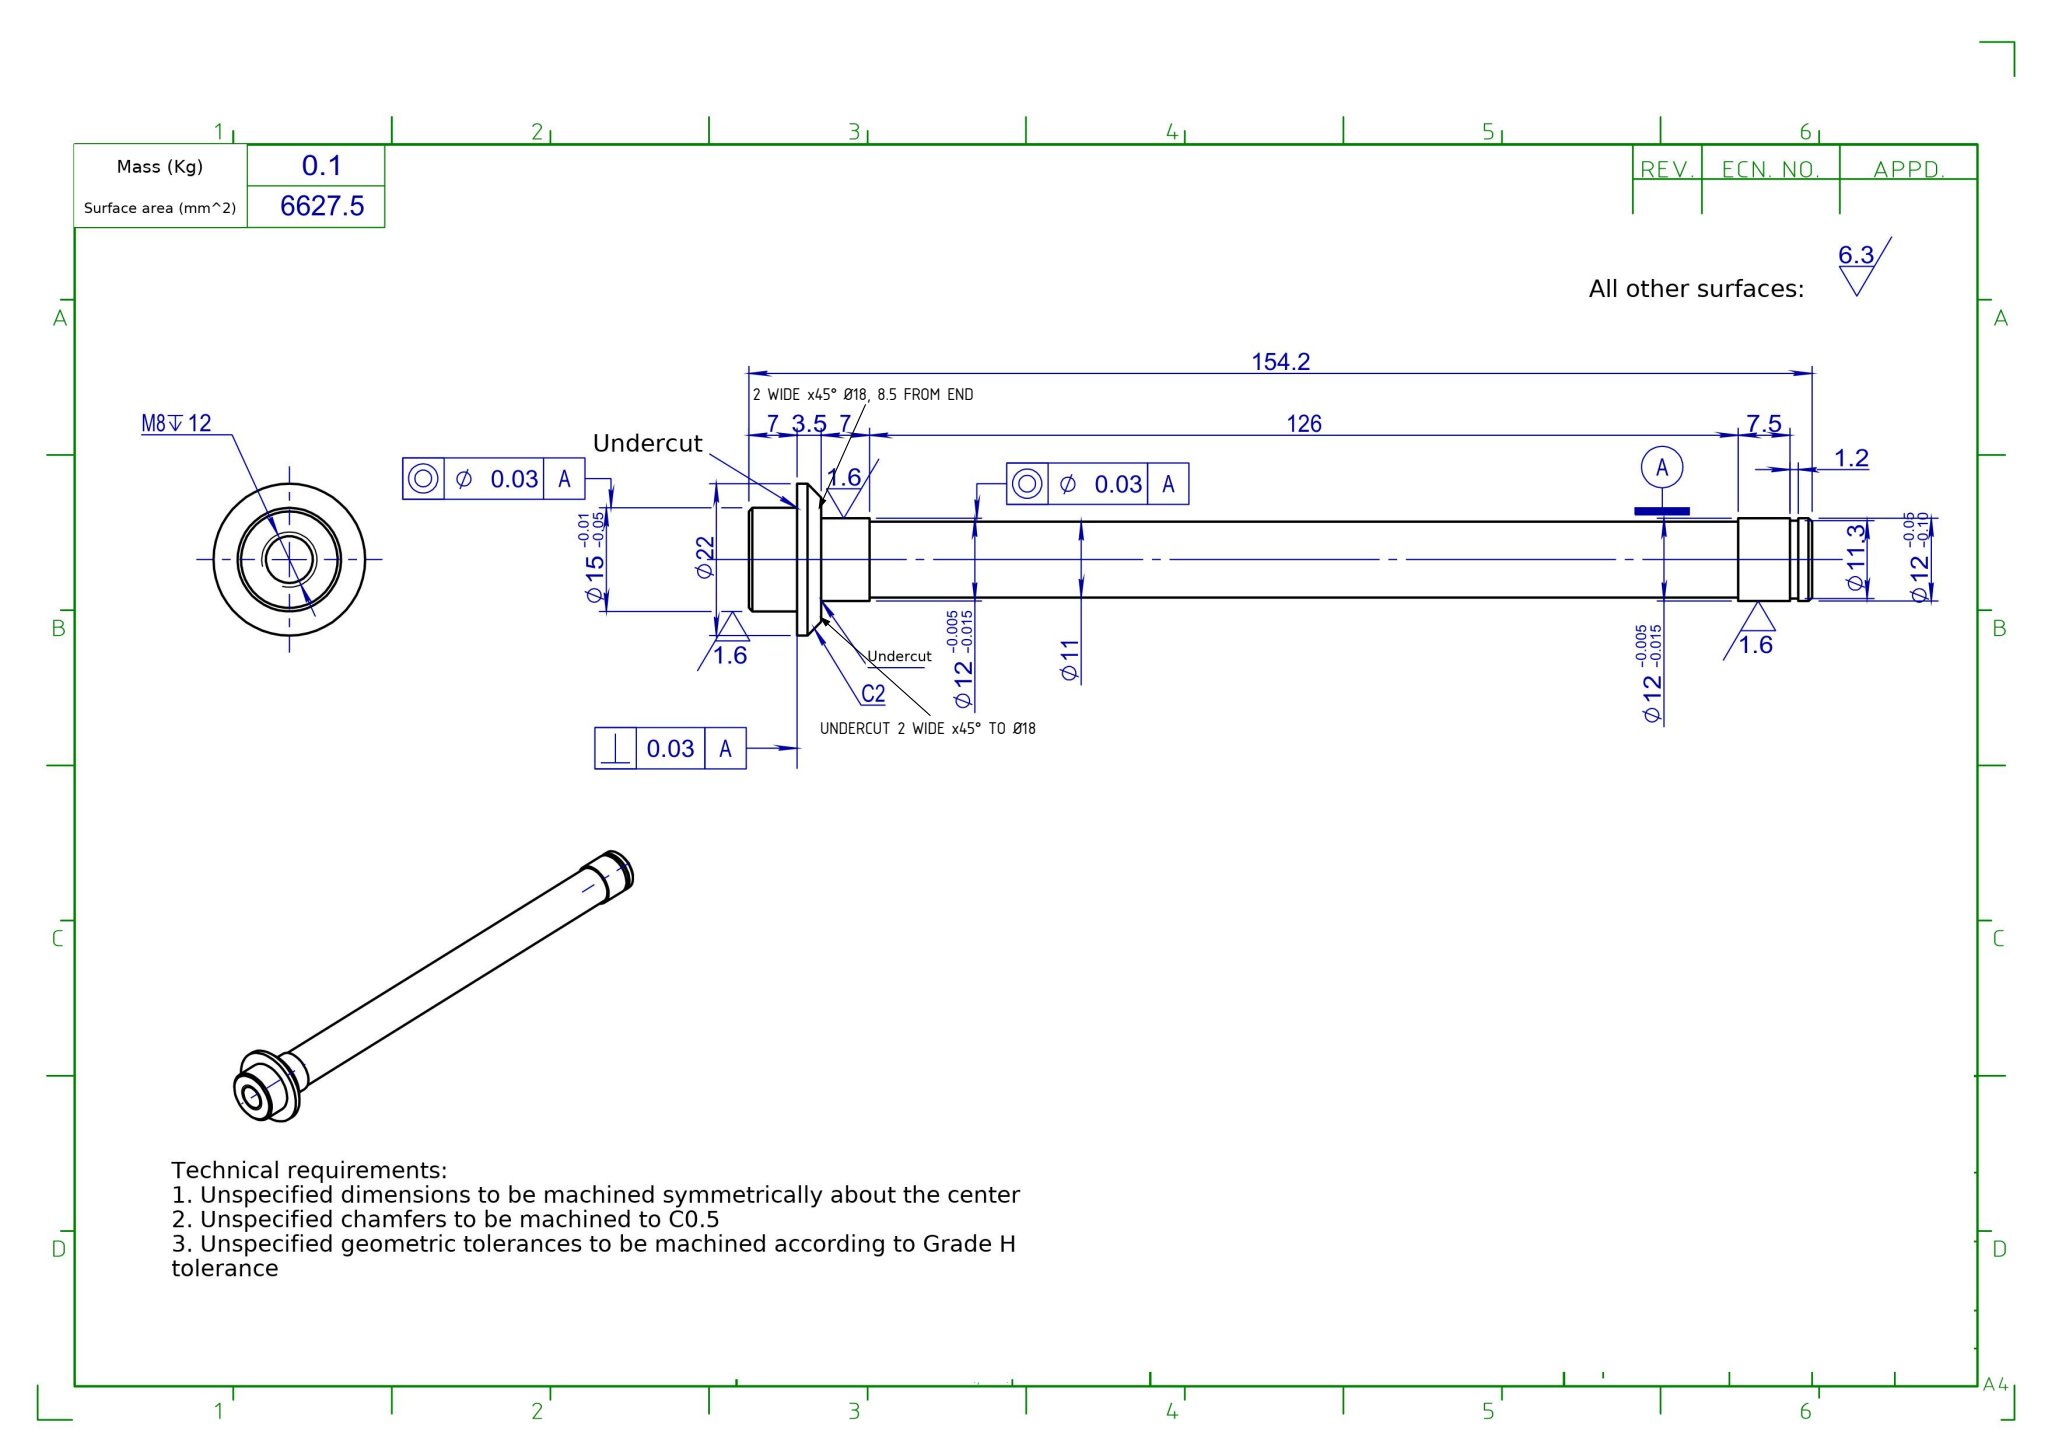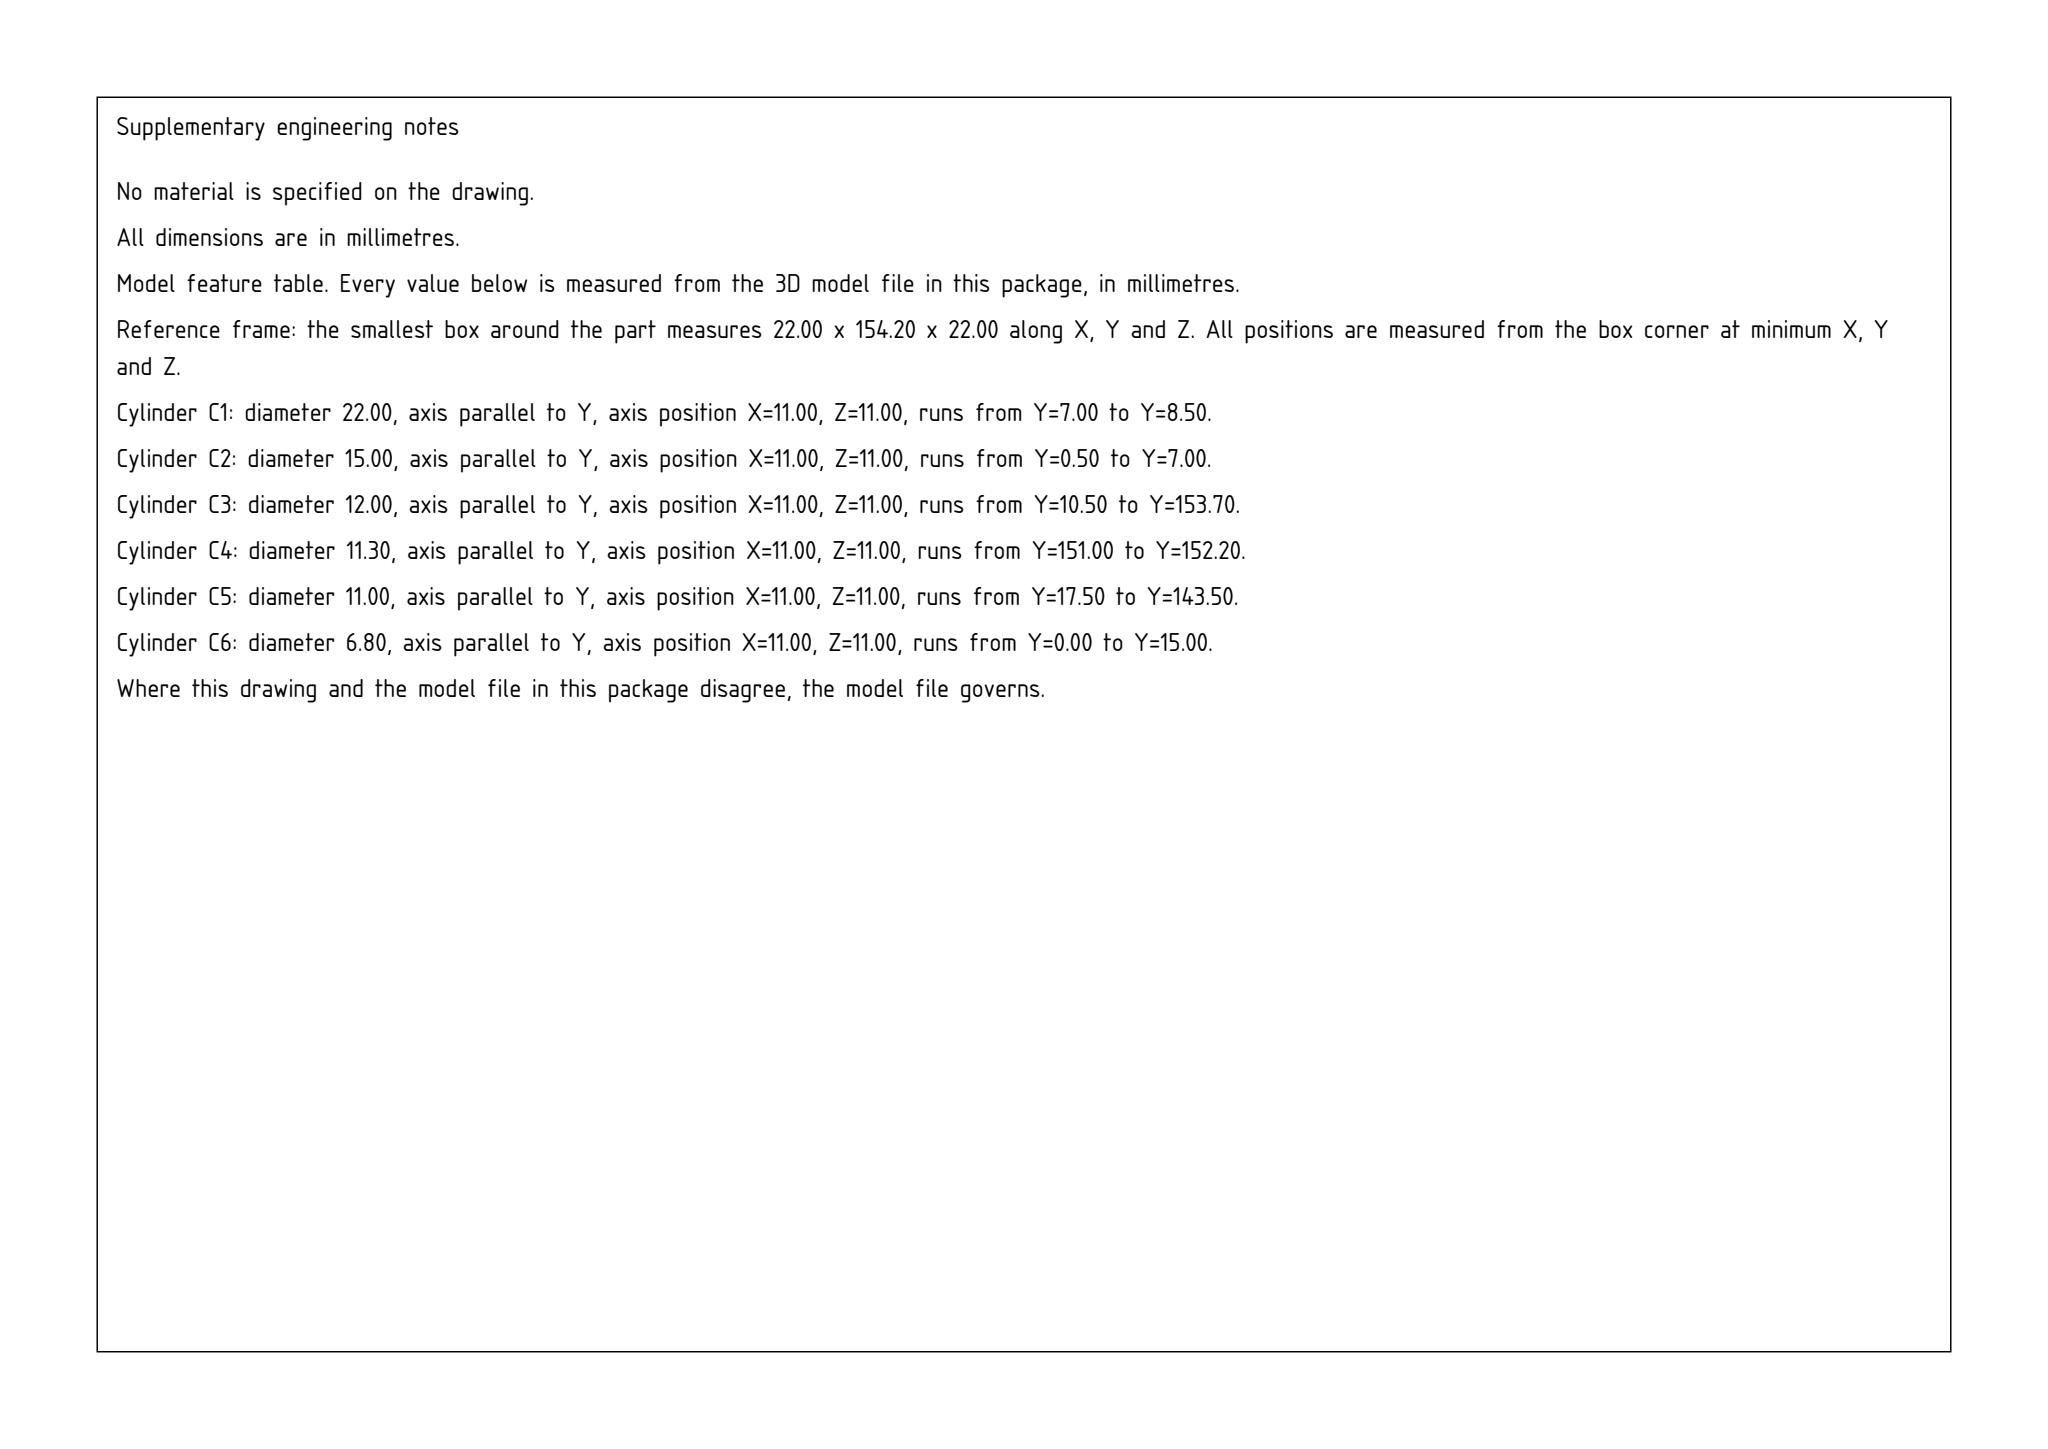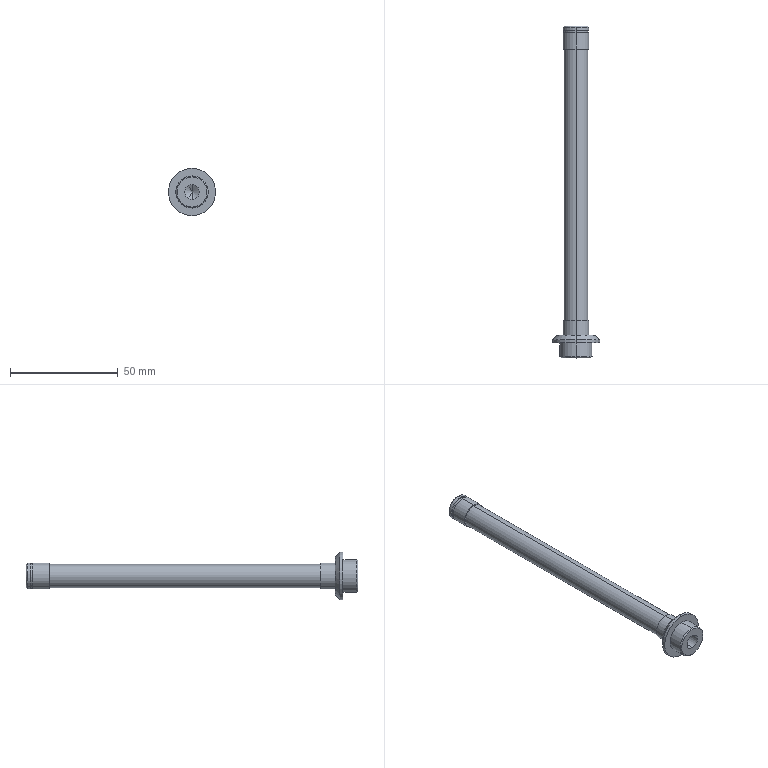Part | SolidWorks | mm | 1 solid | 32 faces | box 22 x 154.2 x 22 mm | volume 15818 mm3 | cylinder 16 | cone 8 | plane 8 | commonest cylinder face diameters 12 x6 6.8 x2 11.3 x2 11 x2 22 x2 15 x2
Drawing notes:
2ND UNDERCUT: 2 WIDE x 45° TO Ø18, STARTS 8.5 FROM LH END | from the solid: 90° cone (45° per side) ref dia 18, y 8.5->10.5, after Ø22 flange ending y=8.5; planar face y=10.5 spans Ø12 to Ø18
UNDERCUT AT Ø22 FLANGE: 2 WIDE x 45°, Ø18 ROOT, TO Ø12 SHLDR | from the solid: Ø22 flange y 7.0-8.5; cone 90° ref Ø18 y 8.5-10.5; Ø12 shaft starts y=10.5 (10.5 = 7 + 3.5 dim chain)
build123d program:
from build123d import *

# Parameters (mm, degrees)
SKETCH1_R             = 7.5
EXTRUDE1_DEPTH        = 7
SKETCH2_R             = 11
EXTRUDE2_DEPTH        = 3.5
SKETCH3_R             = 6
EXTRUDE3_DEPTH        = 7
SKETCH4_R             = 5.5
EXTRUDE4_DEPTH        = 126
SKETCH5_R             = 6
EXTRUDE5_DEPTH        = 7.5
SKETCH6_R             = 5.65
EXTRUDE6_DEPTH        = 1.2
SKETCH7_R             = 6
EXTRUDE7_DEPTH        = 2
M8_TAPPED_HOLE1_D     = 6.8
M8_TAPPED_HOLE1_DEPTH = 15
M8_TAPPED_HOLE1_TIP   = 2.043
CHAMFER1_SIZE         = 2
CHAMFER2_SIZE         = 0.5


with BuildPart() as part:
    # Sketch1 → Extrude1 (new body)
    with BuildSketch(Plane(origin=(0, 0, 0), x_dir=(1, 0, 0), z_dir=(0, 1, 0))):
        with Locations(Location((0, 0, 0), (0, 0, 270))):
            Circle(SKETCH1_R)
    extrude(amount=EXTRUDE1_DEPTH)

    # Sketch2 → Extrude2 (add)
    with BuildSketch(Plane(origin=(0, 7, 0), x_dir=(1, 0, 0), z_dir=(0, 1, 0))):
        with Locations(Location((0, 0, 0), (0, 0, 270))):
            Circle(SKETCH2_R)
    extrude(amount=EXTRUDE2_DEPTH)

    # Sketch3 → Extrude3 (add)
    with BuildSketch(Plane(origin=(0, 10.5, 0), x_dir=(1, 0, 0), z_dir=(0, 1, 0))):
        with Locations(Location((0, 0, 0), (0, 0, 270))):
            Circle(SKETCH3_R)
    extrude(amount=EXTRUDE3_DEPTH)

    # Sketch4 → Extrude4 (add)
    with BuildSketch(Plane(origin=(0, 17.5, 0), x_dir=(1, 0, 0), z_dir=(0, 1, 0))):
        with Locations(Location((0, 0, 0), (0, 0, 270))):
            Circle(SKETCH4_R)
    extrude(amount=EXTRUDE4_DEPTH)

    # Sketch5 → Extrude5 (add)
    with BuildSketch(Plane(origin=(0, 143.5, 0), x_dir=(1, 0, 0), z_dir=(0, 1, 0))):
        with Locations(Location((0, 0, 0), (0, 0, 270))):
            Circle(SKETCH5_R)
    extrude(amount=EXTRUDE5_DEPTH)

    # Sketch6 → Extrude6 (add)
    with BuildSketch(Plane(origin=(0, 151, 0), x_dir=(1, 0, 0), z_dir=(0, 1, 0))):
        with Locations(Location((0, 0, 0), (0, 0, 270))):
            Circle(SKETCH6_R)
    extrude(amount=EXTRUDE6_DEPTH)

    # Sketch7 → Extrude7 (add)
    with BuildSketch(Plane(origin=(0, 152.2, 0), x_dir=(1, 0, 0), z_dir=(0, 1, 0))):
        with Locations(Location((0, 0, 0), (0, 0, 270))):
            Circle(SKETCH7_R)
    extrude(amount=EXTRUDE7_DEPTH)

    # M8 Tapped Hole1
    with Locations(Plane.XZ):
        with Locations((0, 0)):
            Hole(M8_TAPPED_HOLE1_D / 2, depth=M8_TAPPED_HOLE1_DEPTH)
            with Locations((0, 0, -(M8_TAPPED_HOLE1_DEPTH + M8_TAPPED_HOLE1_TIP / 2))):  # 118° drill point
                Cone(0, M8_TAPPED_HOLE1_D / 2, M8_TAPPED_HOLE1_TIP, mode=Mode.SUBTRACT)

    # Chamfer1
    chamfer1_edges = [part.edges().sort_by_distance(p)[0] for p in [
        (0, 10.5, -11),
    ]]
    chamfer(chamfer1_edges, length=CHAMFER1_SIZE)

    # Chamfer2
    chamfer2_edges = [part.edges().sort_by_distance(p)[0] for p in [
        (0, 0, -7.5),
        (0, 154.2, -6),
    ]]
    chamfer(chamfer2_edges, length=CHAMFER2_SIZE)


solid = part.part
STEP:
#1=CARTESIAN_POINT('',(0.,0.,-7.));
#2=VERTEX_POINT('',#1);
#3=CARTESIAN_POINT('',(0.,0.,7.));
#4=VERTEX_POINT('',#3);
#5=CARTESIAN_POINT('',(0.,0.,0.));
#6=DIRECTION('',(0.,-1.,0.));
#7=DIRECTION('',(0.,0.,1.));
#8=AXIS2_PLACEMENT_3D('',#5,#6,#7);
#9=CIRCLE('',#8,7.);
#10=EDGE_CURVE('',#2,#4,#9,.T.);
#11=ORIENTED_EDGE('',*,*,#10,.F.);
#12=CARTESIAN_POINT('',(0.,0.5,-7.5));
#13=VERTEX_POINT('',#12);
#14=CARTESIAN_POINT('',(0.,0.5,-7.5));
#15=DIRECTION('',(0.,0.7071,-0.7071));
#16=VECTOR('',#15,1000.);
#17=LINE('',#14,#16);
#18=EDGE_CURVE('',#2,#13,#17,.T.);
#19=ORIENTED_EDGE('',*,*,#18,.T.);
#20=CARTESIAN_POINT('',(0.,0.5,7.5));
#21=VERTEX_POINT('',#20);
#22=CARTESIAN_POINT('',(0.,0.5,0.));
#23=DIRECTION('',(0.,1.,0.));
#24=DIRECTION('',(0.,0.,1.));
#25=AXIS2_PLACEMENT_3D('',#22,#23,#24);
#26=CIRCLE('',#25,7.5);
#27=EDGE_CURVE('',#21,#13,#26,.T.);
#28=ORIENTED_EDGE('',*,*,#27,.F.);
#29=CARTESIAN_POINT('',(0.,0.5,7.5));
#30=DIRECTION('',(0.,0.7071,0.7071));
#31=VECTOR('',#30,1000.);
#32=LINE('',#29,#31);
#33=EDGE_CURVE('',#4,#21,#32,.T.);
#34=ORIENTED_EDGE('',*,*,#33,.F.);
#35=EDGE_LOOP('',(#11,#19,#28,#34));
#36=FACE_OUTER_BOUND('',#35,.T.);
#37=CARTESIAN_POINT('',(0.,0.5,0.));
#38=DIRECTION('',(0.,1.,0.));
#39=DIRECTION('',(0.,0.,1.));
#40=AXIS2_PLACEMENT_3D('',#37,#38,#39);
#41=CONICAL_SURFACE('',#40,7.5,0.7854);
#42=ADVANCED_FACE('',(#36),#41,.T.);
#43=CARTESIAN_POINT('',(0.,154.2,5.5));
#44=VERTEX_POINT('',#43);
#45=CARTESIAN_POINT('',(0.,154.2,-5.5));
#46=VERTEX_POINT('',#45);
#47=CARTESIAN_POINT('',(0.,154.2,0.));
#48=DIRECTION('',(0.,1.,0.));
#49=DIRECTION('',(0.,0.,1.));
#50=AXIS2_PLACEMENT_3D('',#47,#48,#49);
#51=CIRCLE('',#50,5.5);
#52=EDGE_CURVE('',#44,#46,#51,.T.);
#53=ORIENTED_EDGE('',*,*,#52,.F.);
#54=CARTESIAN_POINT('',(0.,153.7,6.));
#55=VERTEX_POINT('',#54);
#56=CARTESIAN_POINT('',(0.,154.2,5.5));
#57=DIRECTION('',(0.,-0.7071,0.7071));
#58=VECTOR('',#57,1000.);
#59=LINE('',#56,#58);
#60=EDGE_CURVE('',#44,#55,#59,.T.);
#61=ORIENTED_EDGE('',*,*,#60,.T.);
#62=CARTESIAN_POINT('',(0.,153.7,-6.));
#63=VERTEX_POINT('',#62);
#64=CARTESIAN_POINT('',(0.,153.7,0.));
#65=DIRECTION('',(0.,-1.,0.));
#66=DIRECTION('',(0.,0.,1.));
#67=AXIS2_PLACEMENT_3D('',#64,#65,#66);
#68=CIRCLE('',#67,6.);
#69=EDGE_CURVE('',#63,#55,#68,.T.);
#70=ORIENTED_EDGE('',*,*,#69,.F.);
#71=CARTESIAN_POINT('',(0.,154.2,-5.5));
#72=DIRECTION('',(0.,-0.7071,-0.7071));
#73=VECTOR('',#72,1000.);
#74=LINE('',#71,#73);
#75=EDGE_CURVE('',#46,#63,#74,.T.);
#76=ORIENTED_EDGE('',*,*,#75,.F.);
#77=EDGE_LOOP('',(#53,#61,#70,#76));
#78=FACE_OUTER_BOUND('',#77,.T.);
#79=CARTESIAN_POINT('',(0.,154.2,0.));
#80=DIRECTION('',(0.,-1.,0.));
#81=DIRECTION('',(0.,0.,-1.));
#82=AXIS2_PLACEMENT_3D('',#79,#80,#81);
#83=CONICAL_SURFACE('',#82,5.5,0.7854);
#84=ADVANCED_FACE('',(#78),#83,.T.);
#85=CARTESIAN_POINT('',(0.,10.5,9.));
#86=VERTEX_POINT('',#85);
#87=CARTESIAN_POINT('',(0.,10.5,-9.));
#88=VERTEX_POINT('',#87);
#89=CARTESIAN_POINT('',(0.,10.5,0.));
#90=DIRECTION('',(0.,1.,0.));
#91=DIRECTION('',(0.,0.,1.));
#92=AXIS2_PLACEMENT_3D('',#89,#90,#91);
#93=CIRCLE('',#92,9.);
#94=EDGE_CURVE('',#86,#88,#93,.T.);
#95=ORIENTED_EDGE('',*,*,#94,.F.);
#96=CARTESIAN_POINT('',(0.,8.5,11.));
#97=VERTEX_POINT('',#96);
#98=CARTESIAN_POINT('',(0.,10.5,9.));
#99=DIRECTION('',(0.,-0.7071,0.7071));
#100=VECTOR('',#99,1000.);
#101=LINE('',#98,#100);
#102=EDGE_CURVE('',#86,#97,#101,.T.);
#103=ORIENTED_EDGE('',*,*,#102,.T.);
#104=CARTESIAN_POINT('',(0.,8.5,-11.));
#105=VERTEX_POINT('',#104);
#106=CARTESIAN_POINT('',(0.,8.5,0.));
#107=DIRECTION('',(0.,-1.,0.));
#108=DIRECTION('',(0.,0.,1.));
#109=AXIS2_PLACEMENT_3D('',#106,#107,#108);
#110=CIRCLE('',#109,11.);
#111=EDGE_CURVE('',#105,#97,#110,.T.);
#112=ORIENTED_EDGE('',*,*,#111,.F.);
#113=CARTESIAN_POINT('',(0.,10.5,-9.));
#114=DIRECTION('',(0.,-0.7071,-0.7071));
#115=VECTOR('',#114,1000.);
#116=LINE('',#113,#115);
#117=EDGE_CURVE('',#88,#105,#116,.T.);
#118=ORIENTED_EDGE('',*,*,#117,.F.);
#119=EDGE_LOOP('',(#95,#103,#112,#118));
#120=FACE_OUTER_BOUND('',#119,.T.);
#121=CARTESIAN_POINT('',(0.,10.5,0.));
#122=DIRECTION('',(0.,-1.,0.));
#123=DIRECTION('',(0.,0.,-1.));
#124=AXIS2_PLACEMENT_3D('',#121,#122,#123);
#125=CONICAL_SURFACE('',#124,9.,0.7854);
#126=ADVANCED_FACE('',(#120),#125,.T.);
#127=CARTESIAN_POINT('',(-0.,17.043,0.));
#128=VERTEX_POINT('',#127);
#129=CARTESIAN_POINT('',(0.,15.,-3.4));
#130=VERTEX_POINT('',#129);
#131=CARTESIAN_POINT('',(0.,15.,-3.4));
#132=DIRECTION('',(0.,-0.515,-0.8572));
#133=VECTOR('',#132,1000.);
#134=LINE('',#131,#133);
#135=EDGE_CURVE('',#128,#130,#134,.T.);
#136=ORIENTED_EDGE('',*,*,#135,.F.);
#137=CARTESIAN_POINT('',(0.,15.,3.4));
#138=VERTEX_POINT('',#137);
#139=CARTESIAN_POINT('',(0.,15.,3.4));
#140=DIRECTION('',(0.,-0.515,0.8572));
#141=VECTOR('',#140,1000.);
#142=LINE('',#139,#141);
#143=EDGE_CURVE('',#128,#138,#142,.T.);
#144=ORIENTED_EDGE('',*,*,#143,.T.);
#145=CARTESIAN_POINT('',(0.,15.,0.));
#146=DIRECTION('',(0.,-1.,0.));
#147=DIRECTION('',(0.,0.,-1.));
#148=AXIS2_PLACEMENT_3D('',#145,#146,#147);
#149=CIRCLE('',#148,3.4);
#150=EDGE_CURVE('',#138,#130,#149,.T.);
#151=ORIENTED_EDGE('',*,*,#150,.T.);
#152=EDGE_LOOP('',(#136,#144,#151));
#153=FACE_OUTER_BOUND('',#152,.T.);
#154=CARTESIAN_POINT('',(0.,15.,0.));
#155=DIRECTION('',(0.,-1.,0.));
#156=DIRECTION('',(0.,0.,-1.));
#157=AXIS2_PLACEMENT_3D('',#154,#155,#156);
#158=CONICAL_SURFACE('',#157,3.4,1.03);
#159=ADVANCED_FACE('',(#153),#158,.F.);
#160=ORIENTED_EDGE('',*,*,#150,.F.);
#161=CARTESIAN_POINT('',(0.,-0.,3.4));
#162=VERTEX_POINT('',#161);
#163=CARTESIAN_POINT('',(0.,0.,3.4));
#164=DIRECTION('',(0.,-1.,0.));
#165=VECTOR('',#164,1000.);
#166=LINE('',#163,#165);
#167=EDGE_CURVE('',#138,#162,#166,.T.);
#168=ORIENTED_EDGE('',*,*,#167,.T.);
#169=CARTESIAN_POINT('',(0.,-0.,-3.4));
#170=VERTEX_POINT('',#169);
#171=CARTESIAN_POINT('',(0.,-0.,0.));
#172=DIRECTION('',(0.,-1.,0.));
#173=DIRECTION('',(0.,0.,-1.));
#174=AXIS2_PLACEMENT_3D('',#171,#172,#173);
#175=CIRCLE('',#174,3.4);
#176=EDGE_CURVE('',#162,#170,#175,.T.);
#177=ORIENTED_EDGE('',*,*,#176,.T.);
#178=CARTESIAN_POINT('',(0.,0.,-3.4));
#179=DIRECTION('',(0.,-1.,0.));
#180=VECTOR('',#179,1000.);
#181=LINE('',#178,#180);
#182=EDGE_CURVE('',#130,#170,#181,.T.);
#183=ORIENTED_EDGE('',*,*,#182,.F.);
#184=EDGE_LOOP('',(#160,#168,#177,#183));
#185=FACE_OUTER_BOUND('',#184,.T.);
#186=CARTESIAN_POINT('',(0.,0.,0.));
#187=DIRECTION('',(0.,-1.,0.));
#188=DIRECTION('',(0.,0.,-1.));
#189=AXIS2_PLACEMENT_3D('',#186,#187,#188);
#190=CYLINDRICAL_SURFACE('',#189,3.4);
#191=ADVANCED_FACE('',(#185),#190,.F.);
#192=ORIENTED_EDGE('',*,*,#69,.T.);
#193=CARTESIAN_POINT('',(0.,152.2,6.));
#194=VERTEX_POINT('',#193);
#195=CARTESIAN_POINT('',(0.,154.2,6.));
#196=DIRECTION('',(0.,-1.,0.));
#197=VECTOR('',#196,1000.);
#198=LINE('',#195,#197);
#199=EDGE_CURVE('',#55,#194,#198,.T.);
#200=ORIENTED_EDGE('',*,*,#199,.T.);
#201=CARTESIAN_POINT('',(0.,152.2,-6.));
#202=VERTEX_POINT('',#201);
#203=CARTESIAN_POINT('',(0.,152.2,0.));
#204=DIRECTION('',(0.,1.,0.));
#205=DIRECTION('',(0.,0.,1.));
#206=AXIS2_PLACEMENT_3D('',#203,#204,#205);
#207=CIRCLE('',#206,6.);
#208=EDGE_CURVE('',#194,#202,#207,.T.);
#209=ORIENTED_EDGE('',*,*,#208,.T.);
#210=CARTESIAN_POINT('',(0.,154.2,-6.));
#211=DIRECTION('',(0.,-1.,0.));
#212=VECTOR('',#211,1000.);
#213=LINE('',#210,#212);
#214=EDGE_CURVE('',#63,#202,#213,.T.);
#215=ORIENTED_EDGE('',*,*,#214,.F.);
#216=EDGE_LOOP('',(#192,#200,#209,#215));
#217=FACE_OUTER_BOUND('',#216,.T.);
#218=CARTESIAN_POINT('',(0.,154.2,0.));
#219=DIRECTION('',(0.,-1.,0.));
#220=DIRECTION('',(0.,0.,-1.));
#221=AXIS2_PLACEMENT_3D('',#218,#219,#220);
#222=CYLINDRICAL_SURFACE('',#221,6.);
#223=ADVANCED_FACE('',(#217),#222,.T.);
#224=CARTESIAN_POINT('',(0.,152.2,5.65));
#225=VERTEX_POINT('',#224);
#226=CARTESIAN_POINT('',(0.,152.2,-5.65));
#227=VERTEX_POINT('',#226);
#228=CARTESIAN_POINT('',(0.,152.2,0.));
#229=DIRECTION('',(0.,1.,0.));
#230=DIRECTION('',(0.,0.,1.));
#231=AXIS2_PLACEMENT_3D('',#228,#229,#230);
#232=CIRCLE('',#231,5.65);
#233=EDGE_CURVE('',#225,#227,#232,.T.);
#234=ORIENTED_EDGE('',*,*,#233,.F.);
#235=CARTESIAN_POINT('',(0.,151.,5.65));
#236=VERTEX_POINT('',#235);
#237=CARTESIAN_POINT('',(0.,152.2,5.65));
#238=DIRECTION('',(0.,-1.,0.));
#239=VECTOR('',#238,1000.);
#240=LINE('',#237,#239);
#241=EDGE_CURVE('',#225,#236,#240,.T.);
#242=ORIENTED_EDGE('',*,*,#241,.T.);
#243=CARTESIAN_POINT('',(0.,151.,-5.65));
#244=VERTEX_POINT('',#243);
#245=CARTESIAN_POINT('',(0.,151.,0.));
#246=DIRECTION('',(0.,1.,0.));
#247=DIRECTION('',(0.,0.,1.));
#248=AXIS2_PLACEMENT_3D('',#245,#246,#247);
#249=CIRCLE('',#248,5.65);
#250=EDGE_CURVE('',#236,#244,#249,.T.);
#251=ORIENTED_EDGE('',*,*,#250,.T.);
#252=CARTESIAN_POINT('',(0.,152.2,-5.65));
#253=DIRECTION('',(0.,-1.,0.));
#254=VECTOR('',#253,1000.);
#255=LINE('',#252,#254);
#256=EDGE_CURVE('',#227,#244,#255,.T.);
#257=ORIENTED_EDGE('',*,*,#256,.F.);
#258=EDGE_LOOP('',(#234,#242,#251,#257));
#259=FACE_OUTER_BOUND('',#258,.T.);
#260=CARTESIAN_POINT('',(0.,152.2,0.));
#261=DIRECTION('',(0.,-1.,0.));
#262=DIRECTION('',(0.,0.,-1.));
#263=AXIS2_PLACEMENT_3D('',#260,#261,#262);
#264=CYLINDRICAL_SURFACE('',#263,5.65);
#265=ADVANCED_FACE('',(#259),#264,.T.);
#266=CARTESIAN_POINT('',(0.,151.,6.));
#267=VERTEX_POINT('',#266);
#268=CARTESIAN_POINT('',(0.,151.,-6.));
#269=VERTEX_POINT('',#268);
#270=CARTESIAN_POINT('',(0.,151.,0.));
#271=DIRECTION('',(0.,1.,0.));
#272=DIRECTION('',(0.,0.,1.));
#273=AXIS2_PLACEMENT_3D('',#270,#271,#272);
#274=CIRCLE('',#273,6.);
#275=EDGE_CURVE('',#267,#269,#274,.T.);
#276=ORIENTED_EDGE('',*,*,#275,.F.);
#277=CARTESIAN_POINT('',(0.,143.5,6.));
#278=VERTEX_POINT('',#277);
#279=CARTESIAN_POINT('',(0.,151.,6.));
#280=DIRECTION('',(0.,-1.,0.));
#281=VECTOR('',#280,1000.);
#282=LINE('',#279,#281);
#283=EDGE_CURVE('',#267,#278,#282,.T.);
#284=ORIENTED_EDGE('',*,*,#283,.T.);
#285=CARTESIAN_POINT('',(0.,143.5,-6.));
#286=VERTEX_POINT('',#285);
#287=CARTESIAN_POINT('',(0.,143.5,0.));
#288=DIRECTION('',(0.,1.,0.));
#289=DIRECTION('',(0.,0.,1.));
#290=AXIS2_PLACEMENT_3D('',#287,#288,#289);
#291=CIRCLE('',#290,6.);
#292=EDGE_CURVE('',#278,#286,#291,.T.);
#293=ORIENTED_EDGE('',*,*,#292,.T.);
#294=CARTESIAN_POINT('',(0.,151.,-6.));
#295=DIRECTION('',(0.,-1.,0.));
#296=VECTOR('',#295,1000.);
#297=LINE('',#294,#296);
#298=EDGE_CURVE('',#269,#286,#297,.T.);
#299=ORIENTED_EDGE('',*,*,#298,.F.);
#300=EDGE_LOOP('',(#276,#284,#293,#299));
#301=FACE_OUTER_BOUND('',#300,.T.);
#302=CARTESIAN_POINT('',(0.,151.,0.));
#303=DIRECTION('',(0.,-1.,0.));
#304=DIRECTION('',(0.,0.,-1.));
#305=AXIS2_PLACEMENT_3D('',#302,#303,#304);
#306=CYLINDRICAL_SURFACE('',#305,6.);
#307=ADVANCED_FACE('',(#301),#306,.T.);
#308=CARTESIAN_POINT('',(0.,143.5,5.5));
#309=VERTEX_POINT('',#308);
#310=CARTESIAN_POINT('',(0.,143.5,-5.5));
#311=VERTEX_POINT('',#310);
#312=CARTESIAN_POINT('',(0.,143.5,0.));
#313=DIRECTION('',(0.,1.,0.));
#314=DIRECTION('',(0.,0.,1.));
#315=AXIS2_PLACEMENT_3D('',#312,#313,#314);
#316=CIRCLE('',#315,5.5);
#317=EDGE_CURVE('',#309,#311,#316,.T.);
#318=ORIENTED_EDGE('',*,*,#317,.F.);
#319=CARTESIAN_POINT('',(0.,17.5,5.5));
#320=VERTEX_POINT('',#319);
#321=CARTESIAN_POINT('',(0.,143.5,5.5));
#322=DIRECTION('',(0.,-1.,0.));
#323=VECTOR('',#322,1000.);
#324=LINE('',#321,#323);
#325=EDGE_CURVE('',#309,#320,#324,.T.);
#326=ORIENTED_EDGE('',*,*,#325,.T.);
#327=CARTESIAN_POINT('',(0.,17.5,-5.5));
#328=VERTEX_POINT('',#327);
#329=CARTESIAN_POINT('',(0.,17.5,0.));
#330=DIRECTION('',(0.,1.,0.));
#331=DIRECTION('',(0.,0.,1.));
#332=AXIS2_PLACEMENT_3D('',#329,#330,#331);
#333=CIRCLE('',#332,5.5);
#334=EDGE_CURVE('',#320,#328,#333,.T.);
#335=ORIENTED_EDGE('',*,*,#334,.T.);
#336=CARTESIAN_POINT('',(0.,143.5,-5.5));
#337=DIRECTION('',(0.,-1.,0.));
#338=VECTOR('',#337,1000.);
#339=LINE('',#336,#338);
#340=EDGE_CURVE('',#311,#328,#339,.T.);
#341=ORIENTED_EDGE('',*,*,#340,.F.);
#342=EDGE_LOOP('',(#318,#326,#335,#341));
#343=FACE_OUTER_BOUND('',#342,.T.);
#344=CARTESIAN_POINT('',(0.,143.5,0.));
#345=DIRECTION('',(0.,-1.,0.));
#346=DIRECTION('',(0.,0.,-1.));
#347=AXIS2_PLACEMENT_3D('',#344,#345,#346);
#348=CYLINDRICAL_SURFACE('',#347,5.5);
#349=ADVANCED_FACE('',(#343),#348,.T.);
#350=CARTESIAN_POINT('',(0.,17.5,6.));
#351=VERTEX_POINT('',#350);
#352=CARTESIAN_POINT('',(0.,17.5,-6.));
#353=VERTEX_POINT('',#352);
#354=CARTESIAN_POINT('',(0.,17.5,0.));
#355=DIRECTION('',(0.,1.,0.));
#356=DIRECTION('',(0.,0.,1.));
#357=AXIS2_PLACEMENT_3D('',#354,#355,#356);
#358=CIRCLE('',#357,6.);
#359=EDGE_CURVE('',#351,#353,#358,.T.);
#360=ORIENTED_EDGE('',*,*,#359,.F.);
#361=CARTESIAN_POINT('',(0.,10.5,6.));
#362=VERTEX_POINT('',#361);
#363=CARTESIAN_POINT('',(0.,17.5,6.));
#364=DIRECTION('',(0.,-1.,0.));
#365=VECTOR('',#364,1000.);
#366=LINE('',#363,#365);
#367=EDGE_CURVE('',#351,#362,#366,.T.);
#368=ORIENTED_EDGE('',*,*,#367,.T.);
#369=CARTESIAN_POINT('',(0.,10.5,-6.));
#370=VERTEX_POINT('',#369);
#371=CARTESIAN_POINT('',(0.,10.5,0.));
#372=DIRECTION('',(0.,1.,0.));
#373=DIRECTION('',(0.,0.,1.));
#374=AXIS2_PLACEMENT_3D('',#371,#372,#373);
#375=CIRCLE('',#374,6.);
#376=EDGE_CURVE('',#362,#370,#375,.T.);
#377=ORIENTED_EDGE('',*,*,#376,.T.);
#378=CARTESIAN_POINT('',(0.,17.5,-6.));
#379=DIRECTION('',(0.,-1.,0.));
#380=VECTOR('',#379,1000.);
#381=LINE('',#378,#380);
#382=EDGE_CURVE('',#353,#370,#381,.T.);
#383=ORIENTED_EDGE('',*,*,#382,.F.);
#384=EDGE_LOOP('',(#360,#368,#377,#383));
#385=FACE_OUTER_BOUND('',#384,.T.);
#386=CARTESIAN_POINT('',(0.,17.5,0.));
#387=DIRECTION('',(0.,-1.,0.));
#388=DIRECTION('',(0.,0.,-1.));
#389=AXIS2_PLACEMENT_3D('',#386,#387,#388);
#390=CYLINDRICAL_SURFACE('',#389,6.);
#391=ADVANCED_FACE('',(#385),#390,.T.);
#392=ORIENTED_EDGE('',*,*,#111,.T.);
#393=CARTESIAN_POINT('',(0.,7.,11.));
#394=VERTEX_POINT('',#393);
#395=CARTESIAN_POINT('',(0.,10.5,11.));
#396=DIRECTION('',(0.,-1.,0.));
#397=VECTOR('',#396,1000.);
#398=LINE('',#395,#397);
#399=EDGE_CURVE('',#97,#394,#398,.T.);
#400=ORIENTED_EDGE('',*,*,#399,.T.);
#401=CARTESIAN_POINT('',(0.,7.,-11.));
#402=VERTEX_POINT('',#401);
#403=CARTESIAN_POINT('',(0.,7.,0.));
#404=DIRECTION('',(0.,1.,0.));
#405=DIRECTION('',(0.,0.,1.));
#406=AXIS2_PLACEMENT_3D('',#403,#404,#405);
#407=CIRCLE('',#406,11.);
#408=EDGE_CURVE('',#394,#402,#407,.T.);
#409=ORIENTED_EDGE('',*,*,#408,.T.);
#410=CARTESIAN_POINT('',(0.,10.5,-11.));
#411=DIRECTION('',(0.,-1.,0.));
#412=VECTOR('',#411,1000.);
#413=LINE('',#410,#412);
#414=EDGE_CURVE('',#105,#402,#413,.T.);
#415=ORIENTED_EDGE('',*,*,#414,.F.);
#416=EDGE_LOOP('',(#392,#400,#409,#415));
#417=FACE_OUTER_BOUND('',#416,.T.);
#418=CARTESIAN_POINT('',(0.,10.5,0.));
#419=DIRECTION('',(0.,-1.,0.));
#420=DIRECTION('',(0.,0.,-1.));
#421=AXIS2_PLACEMENT_3D('',#418,#419,#420);
#422=CYLINDRICAL_SURFACE('',#421,11.);
#423=ADVANCED_FACE('',(#417),#422,.T.);
#424=CARTESIAN_POINT('',(0.,7.,7.5));
#425=VERTEX_POINT('',#424);
#426=CARTESIAN_POINT('',(0.,7.,-7.5));
#427=VERTEX_POINT('',#426);
#428=CARTESIAN_POINT('',(0.,7.,0.));
#429=DIRECTION('',(0.,1.,0.));
#430=DIRECTION('',(0.,0.,1.));
#431=AXIS2_PLACEMENT_3D('',#428,#429,#430);
#432=CIRCLE('',#431,7.5);
#433=EDGE_CURVE('',#425,#427,#432,.T.);
#434=ORIENTED_EDGE('',*,*,#433,.F.);
#435=CARTESIAN_POINT('',(0.,7.,7.5));
#436=DIRECTION('',(0.,-1.,0.));
#437=VECTOR('',#436,1000.);
#438=LINE('',#435,#437);
#439=EDGE_CURVE('',#425,#21,#438,.T.);
#440=ORIENTED_EDGE('',*,*,#439,.T.);
#441=ORIENTED_EDGE('',*,*,#27,.T.);
#442=CARTESIAN_POINT('',(0.,7.,-7.5));
#443=DIRECTION('',(0.,-1.,0.));
#444=VECTOR('',#443,1000.);
#445=LINE('',#442,#444);
#446=EDGE_CURVE('',#427,#13,#445,.T.);
#447=ORIENTED_EDGE('',*,*,#446,.F.);
#448=EDGE_LOOP('',(#434,#440,#441,#447));
#449=FACE_OUTER_BOUND('',#448,.T.);
#450=CARTESIAN_POINT('',(0.,7.,0.));
#451=DIRECTION('',(0.,-1.,0.));
#452=DIRECTION('',(0.,0.,-1.));
#453=AXIS2_PLACEMENT_3D('',#450,#451,#452);
#454=CYLINDRICAL_SURFACE('',#453,7.5);
#455=ADVANCED_FACE('',(#449),#454,.T.);
#456=CARTESIAN_POINT('',(0.,151.,0.));
#457=DIRECTION('',(0.,1.,0.));
#458=DIRECTION('',(0.,0.,1.));
#459=AXIS2_PLACEMENT_3D('',#456,#457,#458);
#460=CIRCLE('',#459,6.);
#461=EDGE_CURVE('',#269,#267,#460,.T.);
#462=ORIENTED_EDGE('',*,*,#461,.T.);
#463=ORIENTED_EDGE('',*,*,#275,.T.);
#464=EDGE_LOOP('',(#462,#463));
#465=FACE_OUTER_BOUND('',#464,.T.);
#466=CARTESIAN_POINT('',(0.,151.,0.));
#467=DIRECTION('',(0.,1.,0.));
#468=DIRECTION('',(0.,0.,1.));
#469=AXIS2_PLACEMENT_3D('',#466,#467,#468);
#470=CIRCLE('',#469,5.65);
#471=EDGE_CURVE('',#244,#236,#470,.T.);
#472=ORIENTED_EDGE('',*,*,#471,.F.);
#473=ORIENTED_EDGE('',*,*,#250,.F.);
#474=EDGE_LOOP('',(#472,#473));
#475=FACE_BOUND('',#474,.T.);
#476=CARTESIAN_POINT('',(0.,151.,0.));
#477=DIRECTION('',(0.,1.,0.));
#478=DIRECTION('',(0.,0.,1.));
#479=AXIS2_PLACEMENT_3D('',#476,#477,#478);
#480=PLANE('',#479);
#481=ADVANCED_FACE('',(#465,#475),#480,.T.);
#482=CARTESIAN_POINT('',(0.,17.5,0.));
#483=DIRECTION('',(0.,1.,0.));
#484=DIRECTION('',(0.,0.,1.));
#485=AXIS2_PLACEMENT_3D('',#482,#483,#484);
#486=CIRCLE('',#485,6.);
#487=EDGE_CURVE('',#353,#351,#486,.T.);
#488=ORIENTED_EDGE('',*,*,#487,.T.);
#489=ORIENTED_EDGE('',*,*,#359,.T.);
#490=EDGE_LOOP('',(#488,#489));
#491=FACE_OUTER_BOUND('',#490,.T.);
#492=CARTESIAN_POINT('',(0.,17.5,0.));
#493=DIRECTION('',(0.,1.,0.));
#494=DIRECTION('',(0.,0.,1.));
#495=AXIS2_PLACEMENT_3D('',#492,#493,#494);
#496=CIRCLE('',#495,5.5);
#497=EDGE_CURVE('',#328,#320,#496,.T.);
#498=ORIENTED_EDGE('',*,*,#497,.F.);
#499=ORIENTED_EDGE('',*,*,#334,.F.);
#500=EDGE_LOOP('',(#498,#499));
#501=FACE_BOUND('',#500,.T.);
#502=CARTESIAN_POINT('',(0.,17.5,0.));
#503=DIRECTION('',(0.,1.,0.));
#504=DIRECTION('',(0.,0.,1.));
#505=AXIS2_PLACEMENT_3D('',#502,#503,#504);
#506=PLANE('',#505);
#507=ADVANCED_FACE('',(#491,#501),#506,.T.);
#508=CARTESIAN_POINT('',(0.,10.5,0.));
#509=DIRECTION('',(0.,1.,0.));
#510=DIRECTION('',(0.,0.,1.));
#511=AXIS2_PLACEMENT_3D('',#508,#509,#510);
#512=CIRCLE('',#511,9.);
#513=EDGE_CURVE('',#88,#86,#512,.T.);
#514=ORIENTED_EDGE('',*,*,#513,.T.);
#515=ORIENTED_EDGE('',*,*,#94,.T.);
#516=EDGE_LOOP('',(#514,#515));
#517=FACE_OUTER_BOUND('',#516,.T.);
#518=CARTESIAN_POINT('',(0.,10.5,0.));
#519=DIRECTION('',(0.,1.,0.));
#520=DIRECTION('',(0.,0.,1.));
#521=AXIS2_PLACEMENT_3D('',#518,#519,#520);
#522=CIRCLE('',#521,6.);
#523=EDGE_CURVE('',#370,#362,#522,.T.);
#524=ORIENTED_EDGE('',*,*,#523,.F.);
#525=ORIENTED_EDGE('',*,*,#376,.F.);
#526=EDGE_LOOP('',(#524,#525));
#527=FACE_BOUND('',#526,.T.);
#528=CARTESIAN_POINT('',(0.,10.5,0.));
#529=DIRECTION('',(0.,1.,0.));
#530=DIRECTION('',(0.,0.,1.));
#531=AXIS2_PLACEMENT_3D('',#528,#529,#530);
#532=PLANE('',#531);
#533=ADVANCED_FACE('',(#517,#527),#532,.T.);
#534=ORIENTED_EDGE('',*,*,#439,.F.);
#535=CARTESIAN_POINT('',(0.,7.,0.));
#536=DIRECTION('',(0.,1.,0.));
#537=DIRECTION('',(0.,0.,1.));
#538=AXIS2_PLACEMENT_3D('',#535,#536,#537);
#539=CIRCLE('',#538,7.5);
#540=EDGE_CURVE('',#427,#425,#539,.T.);
#541=ORIENTED_EDGE('',*,*,#540,.F.);
#542=ORIENTED_EDGE('',*,*,#446,.T.);
#543=CARTESIAN_POINT('',(0.,0.5,0.));
#544=DIRECTION('',(0.,1.,0.));
#545=DIRECTION('',(0.,0.,1.));
#546=AXIS2_PLACEMENT_3D('',#543,#544,#545);
#547=CIRCLE('',#546,7.5);
#548=EDGE_CURVE('',#13,#21,#547,.T.);
#549=ORIENTED_EDGE('',*,*,#548,.T.);
#550=EDGE_LOOP('',(#534,#541,#542,#549));
#551=FACE_OUTER_BOUND('',#550,.T.);
#552=CARTESIAN_POINT('',(0.,7.,0.));
#553=DIRECTION('',(0.,-1.,0.));
#554=DIRECTION('',(0.,0.,-1.));
#555=AXIS2_PLACEMENT_3D('',#552,#553,#554);
#556=CYLINDRICAL_SURFACE('',#555,7.5);
#557=ADVANCED_FACE('',(#551),#556,.T.);
#558=CARTESIAN_POINT('',(0.,0.,0.));
#559=DIRECTION('',(0.,-1.,0.));
#560=DIRECTION('',(0.,0.,1.));
#561=AXIS2_PLACEMENT_3D('',#558,#559,#560);
#562=CIRCLE('',#561,7.);
#563=EDGE_CURVE('',#4,#2,#562,.T.);
#564=ORIENTED_EDGE('',*,*,#563,.T.);
#565=ORIENTED_EDGE('',*,*,#10,.T.);
#566=EDGE_LOOP('',(#564,#565));
#567=FACE_OUTER_BOUND('',#566,.T.);
#568=CARTESIAN_POINT('',(0.,-0.,0.));
#569=DIRECTION('',(0.,-1.,0.));
#570=DIRECTION('',(0.,0.,-1.));
#571=AXIS2_PLACEMENT_3D('',#568,#569,#570);
#572=CIRCLE('',#571,3.4);
#573=EDGE_CURVE('',#170,#162,#572,.T.);
#574=ORIENTED_EDGE('',*,*,#573,.F.);
#575=ORIENTED_EDGE('',*,*,#176,.F.);
#576=EDGE_LOOP('',(#574,#575));
#577=FACE_BOUND('',#576,.T.);
#578=CARTESIAN_POINT('',(0.,0.,0.));
#579=DIRECTION('',(0.,1.,0.));
#580=DIRECTION('',(0.,0.,1.));
#581=AXIS2_PLACEMENT_3D('',#578,#579,#580);
#582=PLANE('',#581);
#583=ADVANCED_FACE('',(#567,#577),#582,.F.);
#584=CARTESIAN_POINT('',(0.,7.,0.));
#585=DIRECTION('',(0.,1.,0.));
#586=DIRECTION('',(0.,0.,1.));
#587=AXIS2_PLACEMENT_3D('',#584,#585,#586);
#588=CIRCLE('',#587,11.);
#589=EDGE_CURVE('',#402,#394,#588,.T.);
#590=ORIENTED_EDGE('',*,*,#589,.F.);
#591=ORIENTED_EDGE('',*,*,#408,.F.);
#592=EDGE_LOOP('',(#590,#591));
#593=FACE_OUTER_BOUND('',#592,.T.);
#594=ORIENTED_EDGE('',*,*,#540,.T.);
#595=ORIENTED_EDGE('',*,*,#433,.T.);
#596=EDGE_LOOP('',(#594,#595));
#597=FACE_BOUND('',#596,.T.);
#598=CARTESIAN_POINT('',(0.,7.,0.));
#599=DIRECTION('',(0.,1.,0.));
#600=DIRECTION('',(0.,0.,1.));
#601=AXIS2_PLACEMENT_3D('',#598,#599,#600);
#602=PLANE('',#601);
#603=ADVANCED_FACE('',(#593,#597),#602,.F.);
#604=ORIENTED_EDGE('',*,*,#399,.F.);
#605=CARTESIAN_POINT('',(0.,8.5,0.));
#606=DIRECTION('',(0.,-1.,0.));
#607=DIRECTION('',(0.,0.,1.));
#608=AXIS2_PLACEMENT_3D('',#605,#606,#607);
#609=CIRCLE('',#608,11.);
#610=EDGE_CURVE('',#97,#105,#609,.T.);
#611=ORIENTED_EDGE('',*,*,#610,.T.);
#612=ORIENTED_EDGE('',*,*,#414,.T.);
#613=ORIENTED_EDGE('',*,*,#589,.T.);
#614=EDGE_LOOP('',(#604,#611,#612,#613));
#615=FACE_OUTER_BOUND('',#614,.T.);
#616=CARTESIAN_POINT('',(0.,10.5,0.));
#617=DIRECTION('',(0.,-1.,0.));
#618=DIRECTION('',(0.,0.,-1.));
#619=AXIS2_PLACEMENT_3D('',#616,#617,#618);
#620=CYLINDRICAL_SURFACE('',#619,11.);
#621=ADVANCED_FACE('',(#615),#620,.T.);
#622=ORIENTED_EDGE('',*,*,#367,.F.);
#623=ORIENTED_EDGE('',*,*,#487,.F.);
#624=ORIENTED_EDGE('',*,*,#382,.T.);
#625=ORIENTED_EDGE('',*,*,#523,.T.);
#626=EDGE_LOOP('',(#622,#623,#624,#625));
#627=FACE_OUTER_BOUND('',#626,.T.);
#628=CARTESIAN_POINT('',(0.,17.5,0.));
#629=DIRECTION('',(0.,-1.,0.));
#630=DIRECTION('',(0.,0.,-1.));
#631=AXIS2_PLACEMENT_3D('',#628,#629,#630);
#632=CYLINDRICAL_SURFACE('',#631,6.);
#633=ADVANCED_FACE('',(#627),#632,.T.);
#634=ORIENTED_EDGE('',*,*,#325,.F.);
#635=CARTESIAN_POINT('',(0.,143.5,0.));
#636=DIRECTION('',(0.,1.,0.));
#637=DIRECTION('',(0.,0.,1.));
#638=AXIS2_PLACEMENT_3D('',#635,#636,#637);
#639=CIRCLE('',#638,5.5);
#640=EDGE_CURVE('',#311,#309,#639,.T.);
#641=ORIENTED_EDGE('',*,*,#640,.F.);
#642=ORIENTED_EDGE('',*,*,#340,.T.);
#643=ORIENTED_EDGE('',*,*,#497,.T.);
#644=EDGE_LOOP('',(#634,#641,#642,#643));
#645=FACE_OUTER_BOUND('',#644,.T.);
#646=CARTESIAN_POINT('',(0.,143.5,0.));
#647=DIRECTION('',(0.,-1.,0.));
#648=DIRECTION('',(0.,0.,-1.));
#649=AXIS2_PLACEMENT_3D('',#646,#647,#648);
#650=CYLINDRICAL_SURFACE('',#649,5.5);
#651=ADVANCED_FACE('',(#645),#650,.T.);
#652=CARTESIAN_POINT('',(0.,143.5,0.));
#653=DIRECTION('',(0.,1.,0.));
#654=DIRECTION('',(0.,0.,1.));
#655=AXIS2_PLACEMENT_3D('',#652,#653,#654);
#656=CIRCLE('',#655,6.);
#657=EDGE_CURVE('',#286,#278,#656,.T.);
#658=ORIENTED_EDGE('',*,*,#657,.F.);
#659=ORIENTED_EDGE('',*,*,#292,.F.);
#660=EDGE_LOOP('',(#658,#659));
#661=FACE_OUTER_BOUND('',#660,.T.);
#662=ORIENTED_EDGE('',*,*,#640,.T.);
#663=ORIENTED_EDGE('',*,*,#317,.T.);
#664=EDGE_LOOP('',(#662,#663));
#665=FACE_BOUND('',#664,.T.);
#666=CARTESIAN_POINT('',(0.,143.5,0.));
#667=DIRECTION('',(0.,1.,0.));
#668=DIRECTION('',(0.,0.,1.));
#669=AXIS2_PLACEMENT_3D('',#666,#667,#668);
#670=PLANE('',#669);
#671=ADVANCED_FACE('',(#661,#665),#670,.F.);
#672=ORIENTED_EDGE('',*,*,#283,.F.);
#673=ORIENTED_EDGE('',*,*,#461,.F.);
#674=ORIENTED_EDGE('',*,*,#298,.T.);
#675=ORIENTED_EDGE('',*,*,#657,.T.);
#676=EDGE_LOOP('',(#672,#673,#674,#675));
#677=FACE_OUTER_BOUND('',#676,.T.);
#678=CARTESIAN_POINT('',(0.,151.,0.));
#679=DIRECTION('',(0.,-1.,0.));
#680=DIRECTION('',(0.,0.,-1.));
#681=AXIS2_PLACEMENT_3D('',#678,#679,#680);
#682=CYLINDRICAL_SURFACE('',#681,6.);
#683=ADVANCED_FACE('',(#677),#682,.T.);
#684=ORIENTED_EDGE('',*,*,#241,.F.);
#685=CARTESIAN_POINT('',(0.,152.2,0.));
#686=DIRECTION('',(0.,1.,0.));
#687=DIRECTION('',(0.,0.,1.));
#688=AXIS2_PLACEMENT_3D('',#685,#686,#687);
#689=CIRCLE('',#688,5.65);
#690=EDGE_CURVE('',#227,#225,#689,.T.);
#691=ORIENTED_EDGE('',*,*,#690,.F.);
#692=ORIENTED_EDGE('',*,*,#256,.T.);
#693=ORIENTED_EDGE('',*,*,#471,.T.);
#694=EDGE_LOOP('',(#684,#691,#692,#693));
#695=FACE_OUTER_BOUND('',#694,.T.);
#696=CARTESIAN_POINT('',(0.,152.2,0.));
#697=DIRECTION('',(0.,-1.,0.));
#698=DIRECTION('',(0.,0.,-1.));
#699=AXIS2_PLACEMENT_3D('',#696,#697,#698);
#700=CYLINDRICAL_SURFACE('',#699,5.65);
#701=ADVANCED_FACE('',(#695),#700,.T.);
#702=CARTESIAN_POINT('',(0.,152.2,0.));
#703=DIRECTION('',(0.,1.,0.));
#704=DIRECTION('',(0.,0.,1.));
#705=AXIS2_PLACEMENT_3D('',#702,#703,#704);
#706=CIRCLE('',#705,6.);
#707=EDGE_CURVE('',#202,#194,#706,.T.);
#708=ORIENTED_EDGE('',*,*,#707,.F.);
#709=ORIENTED_EDGE('',*,*,#208,.F.);
#710=EDGE_LOOP('',(#708,#709));
#711=FACE_OUTER_BOUND('',#710,.T.);
#712=ORIENTED_EDGE('',*,*,#690,.T.);
#713=ORIENTED_EDGE('',*,*,#233,.T.);
#714=EDGE_LOOP('',(#712,#713));
#715=FACE_BOUND('',#714,.T.);
#716=CARTESIAN_POINT('',(0.,152.2,0.));
#717=DIRECTION('',(0.,1.,0.));
#718=DIRECTION('',(0.,0.,1.));
#719=AXIS2_PLACEMENT_3D('',#716,#717,#718);
#720=PLANE('',#719);
#721=ADVANCED_FACE('',(#711,#715),#720,.F.);
#722=ORIENTED_EDGE('',*,*,#199,.F.);
#723=CARTESIAN_POINT('',(0.,153.7,0.));
#724=DIRECTION('',(0.,-1.,0.));
#725=DIRECTION('',(0.,0.,1.));
#726=AXIS2_PLACEMENT_3D('',#723,#724,#725);
#727=CIRCLE('',#726,6.);
#728=EDGE_CURVE('',#55,#63,#727,.T.);
#729=ORIENTED_EDGE('',*,*,#728,.T.);
#730=ORIENTED_EDGE('',*,*,#214,.T.);
#731=ORIENTED_EDGE('',*,*,#707,.T.);
#732=EDGE_LOOP('',(#722,#729,#730,#731));
#733=FACE_OUTER_BOUND('',#732,.T.);
#734=CARTESIAN_POINT('',(0.,154.2,0.));
#735=DIRECTION('',(0.,-1.,0.));
#736=DIRECTION('',(0.,0.,-1.));
#737=AXIS2_PLACEMENT_3D('',#734,#735,#736);
#738=CYLINDRICAL_SURFACE('',#737,6.);
#739=ADVANCED_FACE('',(#733),#738,.T.);
#740=CARTESIAN_POINT('',(0.,154.2,0.));
#741=DIRECTION('',(0.,1.,0.));
#742=DIRECTION('',(0.,0.,1.));
#743=AXIS2_PLACEMENT_3D('',#740,#741,#742);
#744=CIRCLE('',#743,5.5);
#745=EDGE_CURVE('',#46,#44,#744,.T.);
#746=ORIENTED_EDGE('',*,*,#745,.T.);
#747=ORIENTED_EDGE('',*,*,#52,.T.);
#748=EDGE_LOOP('',(#746,#747));
#749=FACE_OUTER_BOUND('',#748,.T.);
#750=CARTESIAN_POINT('',(0.,154.2,0.));
#751=DIRECTION('',(0.,1.,0.));
#752=DIRECTION('',(0.,0.,1.));
#753=AXIS2_PLACEMENT_3D('',#750,#751,#752);
#754=PLANE('',#753);
#755=ADVANCED_FACE('',(#749),#754,.T.);
#756=ORIENTED_EDGE('',*,*,#167,.F.);
#757=CARTESIAN_POINT('',(0.,15.,0.));
#758=DIRECTION('',(0.,-1.,0.));
#759=DIRECTION('',(0.,0.,-1.));
#760=AXIS2_PLACEMENT_3D('',#757,#758,#759);
#761=CIRCLE('',#760,3.4);
#762=EDGE_CURVE('',#130,#138,#761,.T.);
#763=ORIENTED_EDGE('',*,*,#762,.F.);
#764=ORIENTED_EDGE('',*,*,#182,.T.);
#765=ORIENTED_EDGE('',*,*,#573,.T.);
#766=EDGE_LOOP('',(#756,#763,#764,#765));
#767=FACE_OUTER_BOUND('',#766,.T.);
#768=CARTESIAN_POINT('',(0.,0.,0.));
#769=DIRECTION('',(0.,-1.,0.));
#770=DIRECTION('',(0.,0.,-1.));
#771=AXIS2_PLACEMENT_3D('',#768,#769,#770);
#772=CYLINDRICAL_SURFACE('',#771,3.4);
#773=ADVANCED_FACE('',(#767),#772,.F.);
#774=ORIENTED_EDGE('',*,*,#143,.F.);
#775=ORIENTED_EDGE('',*,*,#135,.T.);
#776=ORIENTED_EDGE('',*,*,#762,.T.);
#777=EDGE_LOOP('',(#774,#775,#776));
#778=FACE_OUTER_BOUND('',#777,.T.);
#779=CARTESIAN_POINT('',(0.,15.,0.));
#780=DIRECTION('',(0.,-1.,0.));
#781=DIRECTION('',(0.,0.,-1.));
#782=AXIS2_PLACEMENT_3D('',#779,#780,#781);
#783=CONICAL_SURFACE('',#782,3.4,1.03);
#784=ADVANCED_FACE('',(#778),#783,.F.);
#785=ORIENTED_EDGE('',*,*,#102,.F.);
#786=ORIENTED_EDGE('',*,*,#513,.F.);
#787=ORIENTED_EDGE('',*,*,#117,.T.);
#788=ORIENTED_EDGE('',*,*,#610,.F.);
#789=EDGE_LOOP('',(#785,#786,#787,#788));
#790=FACE_OUTER_BOUND('',#789,.T.);
#791=CARTESIAN_POINT('',(0.,10.5,0.));
#792=DIRECTION('',(0.,-1.,0.));
#793=DIRECTION('',(0.,0.,-1.));
#794=AXIS2_PLACEMENT_3D('',#791,#792,#793);
#795=CONICAL_SURFACE('',#794,9.,0.7854);
#796=ADVANCED_FACE('',(#790),#795,.T.);
#797=ORIENTED_EDGE('',*,*,#60,.F.);
#798=ORIENTED_EDGE('',*,*,#745,.F.);
#799=ORIENTED_EDGE('',*,*,#75,.T.);
#800=ORIENTED_EDGE('',*,*,#728,.F.);
#801=EDGE_LOOP('',(#797,#798,#799,#800));
#802=FACE_OUTER_BOUND('',#801,.T.);
#803=CARTESIAN_POINT('',(0.,154.2,0.));
#804=DIRECTION('',(0.,-1.,0.));
#805=DIRECTION('',(0.,0.,-1.));
#806=AXIS2_PLACEMENT_3D('',#803,#804,#805);
#807=CONICAL_SURFACE('',#806,5.5,0.7854);
#808=ADVANCED_FACE('',(#802),#807,.T.);
#809=ORIENTED_EDGE('',*,*,#18,.F.);
#810=ORIENTED_EDGE('',*,*,#563,.F.);
#811=ORIENTED_EDGE('',*,*,#33,.T.);
#812=ORIENTED_EDGE('',*,*,#548,.F.);
#813=EDGE_LOOP('',(#809,#810,#811,#812));
#814=FACE_OUTER_BOUND('',#813,.T.);
#815=CARTESIAN_POINT('',(0.,0.5,0.));
#816=DIRECTION('',(0.,1.,0.));
#817=DIRECTION('',(0.,0.,1.));
#818=AXIS2_PLACEMENT_3D('',#815,#816,#817);
#819=CONICAL_SURFACE('',#818,7.5,0.7854);
#820=ADVANCED_FACE('',(#814),#819,.T.);
#821=CLOSED_SHELL('',(#42,#84,#126,#159,#191,#223,#265,#307,#349,#391,#423,#455,#481,#507,#533,#557,#583,#603,#621,#633,#651,#671,#683,#701,#721,#739,#755,#773,#784,#796,#808,#820));
#822=MANIFOLD_SOLID_BREP('',#821);
#823=CARTESIAN_POINT('',(0.,0.,0.));
#824=DIRECTION('',(0.,0.,1.));
#825=DIRECTION('',(1.,0.,0.));
#826=AXIS2_PLACEMENT_3D('',#823,#824,#825);
#827=(LENGTH_UNIT()NAMED_UNIT(*)SI_UNIT(.MILLI.,.METRE.));
#828=UNCERTAINTY_MEASURE_WITH_UNIT(LENGTH_MEASURE(0.00001),#827,'','');
#829=(NAMED_UNIT(*)PLANE_ANGLE_UNIT()SI_UNIT($,.RADIAN.));
#830=(NAMED_UNIT(*)SI_UNIT($,.STERADIAN.)SOLID_ANGLE_UNIT());
#831=(GEOMETRIC_REPRESENTATION_CONTEXT(3)GLOBAL_UNCERTAINTY_ASSIGNED_CONTEXT((#828))GLOBAL_UNIT_ASSIGNED_CONTEXT((#827,#829,#830))REPRESENTATION_CONTEXT('',''));
#832=ADVANCED_BREP_SHAPE_REPRESENTATION('',(#822,#826),#831);